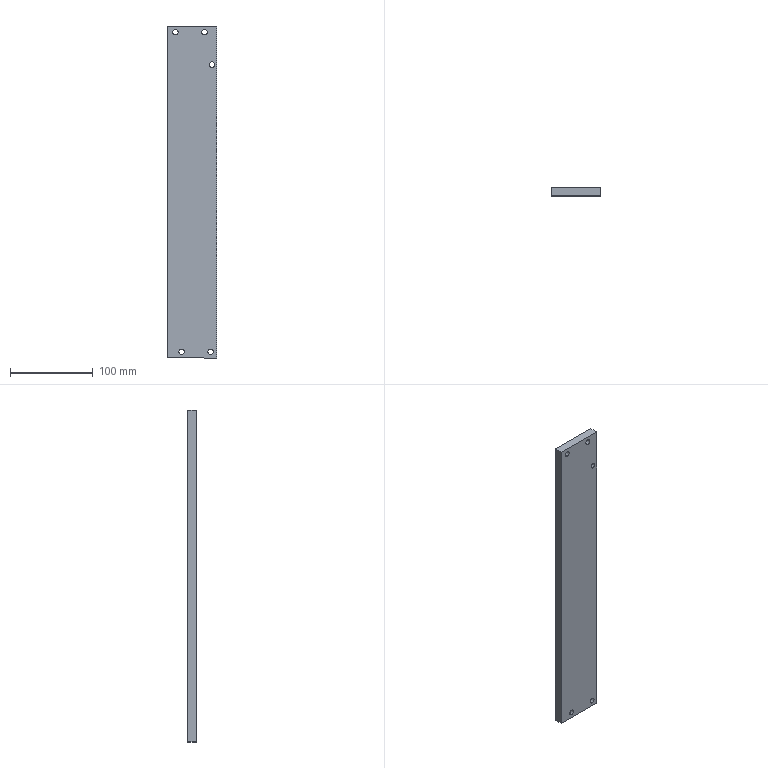Component | SolidWorks | CTM-HVS-42-02-30-1 | 1 solid | 16 faces | box 60 x 10 x 400 mm | volume 238289 mm3 | cylinder 10 | plane 6 | commonest cylinder face diameters 6.6 x10 | material Q235A
build123d program:
from build123d import *

# Parameters (mm, degrees)
SKETCH1_W                      = 400
SKETCH1_H                      = 60
EXTRUDE1_DEPTH                 = 5
SKETCH2_R                      = 3.3
EXTRUDE2_DEPTH                 = 203.485
LPATTERN1_COUNT                = 2
LPATTERN1_PITCH                = 35
M6_CLEARANCE_HOLE1_D           = 6.6
M6_CLEARANCE_HOLE1_DEPTH       = 50
M6_CLEARANCE_HOLE1_TIP         = 1.983
F_6_6_6_6_DIAMETER_HOLE1_D     = 6.6
F_6_6_6_6_DIAMETER_HOLE1_DEPTH = 30
F_6_6_6_6_DIAMETER_HOLE1_TIP   = 1.983


with BuildPart() as part:
    # Sketch1 → Extrude1 (new, symmetric)
    with BuildSketch(Plane.XY):
        Rectangle(SKETCH1_W, SKETCH1_H)
    extrude(amount=EXTRUDE1_DEPTH, both=True)

    # Sketch2 → Extrude2 (cut, through all)
    with BuildSketch(Plane.XY.offset(5)):
        with Locations((-192.5, 20)):
            Circle(SKETCH2_R)
    extrude2 = extrude(amount=-EXTRUDE2_DEPTH, mode=Mode.SUBTRACT)

    # LPattern1: Extrude2 ×2
    with Locations(*[(0, -i * LPATTERN1_PITCH, 0) for i in range(1, LPATTERN1_COUNT)]):
        add(extrude2, mode=Mode.SUBTRACT)

    # M6 Clearance Hole1
    with Locations(Plane.XY.offset(5)):
        with Locations((192.5, 12.5), (192.5, -22.5)):
            Hole(M6_CLEARANCE_HOLE1_D / 2, depth=M6_CLEARANCE_HOLE1_DEPTH)
            with Locations((0, 0, -(M6_CLEARANCE_HOLE1_DEPTH + M6_CLEARANCE_HOLE1_TIP / 2))):  # 118° drill point
                Cone(0, M6_CLEARANCE_HOLE1_D / 2, M6_CLEARANCE_HOLE1_TIP, mode=Mode.SUBTRACT)

    # 6.6 _6.6_ Diameter Hole1
    with Locations(Plane.XY.offset(5)):
        with Locations((-153.5, -24)):
            Hole(F_6_6_6_6_DIAMETER_HOLE1_D / 2, depth=F_6_6_6_6_DIAMETER_HOLE1_DEPTH)
            with Locations((0, 0, -(F_6_6_6_6_DIAMETER_HOLE1_DEPTH + F_6_6_6_6_DIAMETER_HOLE1_TIP / 2))):  # 118° drill point
                Cone(0, F_6_6_6_6_DIAMETER_HOLE1_D / 2, F_6_6_6_6_DIAMETER_HOLE1_TIP, mode=Mode.SUBTRACT)


solid = part.part

# Placed as in the assembly
solid = solid.moved(Location((-292.307, 87.443, 192.5), (-90, 0, 90)))
STEP:
#1=COLOUR_RGB('',0.7922,0.8196,0.9333);
#2=FILL_AREA_STYLE_COLOUR('',#1);
#3=FILL_AREA_STYLE('',(#2));
#4=SURFACE_STYLE_FILL_AREA(#3);
#5=SURFACE_SIDE_STYLE('',(#4));
#6=SURFACE_STYLE_USAGE(.BOTH.,#5);
#7=PRESENTATION_STYLE_ASSIGNMENT((#6));
#8=CARTESIAN_POINT('',(-10.563,3.246,13.752));
#9=VERTEX_POINT('',#8);
#10=CARTESIAN_POINT('',(-10.563,3.246,13.492));
#11=VERTEX_POINT('',#10);
#12=CARTESIAN_POINT('',(-10.563,3.246,13.622));
#13=DIRECTION('',(0.,1.,-0.));
#14=DIRECTION('',(0.,0.,-1.));
#15=AXIS2_PLACEMENT_3D('',#12,#13,#14);
#16=CIRCLE('',#15,0.1299);
#17=EDGE_CURVE('',#9,#11,#16,.T.);
#18=ORIENTED_EDGE('',*,*,#17,.F.);
#19=CARTESIAN_POINT('',(-10.563,3.639,13.752));
#20=VERTEX_POINT('',#19);
#21=CARTESIAN_POINT('',(-10.563,3.639,13.752));
#22=DIRECTION('',(0.,1.,-0.));
#23=VECTOR('',#22,39.37);
#24=LINE('',#21,#23);
#25=EDGE_CURVE('',#9,#20,#24,.T.);
#26=ORIENTED_EDGE('',*,*,#25,.T.);
#27=CARTESIAN_POINT('',(-10.563,3.639,13.492));
#28=VERTEX_POINT('',#27);
#29=CARTESIAN_POINT('',(-10.563,3.639,13.622));
#30=DIRECTION('',(0.,1.,-0.));
#31=DIRECTION('',(0.,0.,-1.));
#32=AXIS2_PLACEMENT_3D('',#29,#30,#31);
#33=CIRCLE('',#32,0.1299);
#34=EDGE_CURVE('',#20,#28,#33,.T.);
#35=ORIENTED_EDGE('',*,*,#34,.T.);
#36=CARTESIAN_POINT('',(-10.563,3.639,13.492));
#37=DIRECTION('',(0.,1.,-0.));
#38=VECTOR('',#37,39.37);
#39=LINE('',#36,#38);
#40=EDGE_CURVE('',#11,#28,#39,.T.);
#41=ORIENTED_EDGE('',*,*,#40,.F.);
#42=EDGE_LOOP('',(#18,#26,#35,#41));
#43=FACE_OUTER_BOUND('',#42,.T.);
#44=CARTESIAN_POINT('',(-10.563,3.639,13.622));
#45=DIRECTION('',(0.,1.,-0.));
#46=DIRECTION('',(0.,0.,-1.));
#47=AXIS2_PLACEMENT_3D('',#44,#45,#46);
#48=CYLINDRICAL_SURFACE('',#47,0.1299);
#49=ADVANCED_FACE('',(#43),#48,.F.);
#50=CARTESIAN_POINT('',(-12.,3.246,0.1299));
#51=VERTEX_POINT('',#50);
#52=CARTESIAN_POINT('',(-12.,3.246,-0.1299));
#53=VERTEX_POINT('',#52);
#54=CARTESIAN_POINT('',(-12.,3.246,0.));
#55=DIRECTION('',(0.,1.,-0.));
#56=DIRECTION('',(0.,0.,-1.));
#57=AXIS2_PLACEMENT_3D('',#54,#55,#56);
#58=CIRCLE('',#57,0.1299);
#59=EDGE_CURVE('',#51,#53,#58,.T.);
#60=ORIENTED_EDGE('',*,*,#59,.F.);
#61=CARTESIAN_POINT('',(-12.,3.639,0.1299));
#62=VERTEX_POINT('',#61);
#63=CARTESIAN_POINT('',(-12.,3.639,0.1299));
#64=DIRECTION('',(0.,1.,-0.));
#65=VECTOR('',#64,39.37);
#66=LINE('',#63,#65);
#67=EDGE_CURVE('',#51,#62,#66,.T.);
#68=ORIENTED_EDGE('',*,*,#67,.T.);
#69=CARTESIAN_POINT('',(-12.,3.639,-0.1299));
#70=VERTEX_POINT('',#69);
#71=CARTESIAN_POINT('',(-12.,3.639,0.));
#72=DIRECTION('',(0.,1.,-0.));
#73=DIRECTION('',(0.,0.,-1.));
#74=AXIS2_PLACEMENT_3D('',#71,#72,#73);
#75=CIRCLE('',#74,0.1299);
#76=EDGE_CURVE('',#62,#70,#75,.T.);
#77=ORIENTED_EDGE('',*,*,#76,.T.);
#78=CARTESIAN_POINT('',(-12.,3.639,-0.1299));
#79=DIRECTION('',(0.,1.,-0.));
#80=VECTOR('',#79,39.37);
#81=LINE('',#78,#80);
#82=EDGE_CURVE('',#53,#70,#81,.T.);
#83=ORIENTED_EDGE('',*,*,#82,.F.);
#84=EDGE_LOOP('',(#60,#68,#77,#83));
#85=FACE_OUTER_BOUND('',#84,.T.);
#86=CARTESIAN_POINT('',(-12.,3.639,0.));
#87=DIRECTION('',(0.,1.,-0.));
#88=DIRECTION('',(0.,0.,-1.));
#89=AXIS2_PLACEMENT_3D('',#86,#87,#88);
#90=CYLINDRICAL_SURFACE('',#89,0.1299);
#91=ADVANCED_FACE('',(#85),#90,.F.);
#92=CARTESIAN_POINT('',(-10.622,3.246,0.1299));
#93=VERTEX_POINT('',#92);
#94=CARTESIAN_POINT('',(-10.622,3.246,-0.1299));
#95=VERTEX_POINT('',#94);
#96=CARTESIAN_POINT('',(-10.622,3.246,0.));
#97=DIRECTION('',(0.,1.,-0.));
#98=DIRECTION('',(0.,0.,-1.));
#99=AXIS2_PLACEMENT_3D('',#96,#97,#98);
#100=CIRCLE('',#99,0.1299);
#101=EDGE_CURVE('',#93,#95,#100,.T.);
#102=ORIENTED_EDGE('',*,*,#101,.F.);
#103=CARTESIAN_POINT('',(-10.622,3.639,0.1299));
#104=VERTEX_POINT('',#103);
#105=CARTESIAN_POINT('',(-10.622,3.639,0.1299));
#106=DIRECTION('',(0.,1.,-0.));
#107=VECTOR('',#106,39.37);
#108=LINE('',#105,#107);
#109=EDGE_CURVE('',#93,#104,#108,.T.);
#110=ORIENTED_EDGE('',*,*,#109,.T.);
#111=CARTESIAN_POINT('',(-10.622,3.639,-0.1299));
#112=VERTEX_POINT('',#111);
#113=CARTESIAN_POINT('',(-10.622,3.639,0.));
#114=DIRECTION('',(0.,1.,-0.));
#115=DIRECTION('',(0.,0.,-1.));
#116=AXIS2_PLACEMENT_3D('',#113,#114,#115);
#117=CIRCLE('',#116,0.1299);
#118=EDGE_CURVE('',#104,#112,#117,.T.);
#119=ORIENTED_EDGE('',*,*,#118,.T.);
#120=CARTESIAN_POINT('',(-10.622,3.639,-0.1299));
#121=DIRECTION('',(0.,1.,-0.));
#122=VECTOR('',#121,39.37);
#123=LINE('',#120,#122);
#124=EDGE_CURVE('',#95,#112,#123,.T.);
#125=ORIENTED_EDGE('',*,*,#124,.F.);
#126=EDGE_LOOP('',(#102,#110,#119,#125));
#127=FACE_OUTER_BOUND('',#126,.T.);
#128=CARTESIAN_POINT('',(-10.622,3.639,0.));
#129=DIRECTION('',(0.,1.,-0.));
#130=DIRECTION('',(0.,0.,-1.));
#131=AXIS2_PLACEMENT_3D('',#128,#129,#130);
#132=CYLINDRICAL_SURFACE('',#131,0.1299);
#133=ADVANCED_FACE('',(#127),#132,.F.);
#134=CARTESIAN_POINT('',(-10.918,3.246,15.287));
#135=VERTEX_POINT('',#134);
#136=CARTESIAN_POINT('',(-10.918,3.246,15.028));
#137=VERTEX_POINT('',#136);
#138=CARTESIAN_POINT('',(-10.918,3.246,15.157));
#139=DIRECTION('',(0.,1.,-0.));
#140=DIRECTION('',(0.,0.,-1.));
#141=AXIS2_PLACEMENT_3D('',#138,#139,#140);
#142=CIRCLE('',#141,0.1299);
#143=EDGE_CURVE('',#135,#137,#142,.T.);
#144=ORIENTED_EDGE('',*,*,#143,.F.);
#145=CARTESIAN_POINT('',(-10.918,3.639,15.287));
#146=VERTEX_POINT('',#145);
#147=CARTESIAN_POINT('',(-10.918,3.246,15.287));
#148=DIRECTION('',(0.,1.,-0.));
#149=VECTOR('',#148,39.37);
#150=LINE('',#147,#149);
#151=EDGE_CURVE('',#135,#146,#150,.T.);
#152=ORIENTED_EDGE('',*,*,#151,.T.);
#153=CARTESIAN_POINT('',(-10.918,3.639,15.028));
#154=VERTEX_POINT('',#153);
#155=CARTESIAN_POINT('',(-10.918,3.639,15.157));
#156=DIRECTION('',(0.,1.,-0.));
#157=DIRECTION('',(0.,0.,-1.));
#158=AXIS2_PLACEMENT_3D('',#155,#156,#157);
#159=CIRCLE('',#158,0.1299);
#160=EDGE_CURVE('',#146,#154,#159,.T.);
#161=ORIENTED_EDGE('',*,*,#160,.T.);
#162=CARTESIAN_POINT('',(-10.918,3.246,15.028));
#163=DIRECTION('',(0.,1.,-0.));
#164=VECTOR('',#163,39.37);
#165=LINE('',#162,#164);
#166=EDGE_CURVE('',#137,#154,#165,.T.);
#167=ORIENTED_EDGE('',*,*,#166,.F.);
#168=EDGE_LOOP('',(#144,#152,#161,#167));
#169=FACE_OUTER_BOUND('',#168,.T.);
#170=CARTESIAN_POINT('',(-10.918,3.246,15.157));
#171=DIRECTION('',(0.,1.,-0.));
#172=DIRECTION('',(0.,0.,-1.));
#173=AXIS2_PLACEMENT_3D('',#170,#171,#172);
#174=CYLINDRICAL_SURFACE('',#173,0.1299);
#175=ADVANCED_FACE('',(#169),#174,.F.);
#176=CARTESIAN_POINT('',(-12.296,3.246,15.287));
#177=VERTEX_POINT('',#176);
#178=CARTESIAN_POINT('',(-12.296,3.246,15.028));
#179=VERTEX_POINT('',#178);
#180=CARTESIAN_POINT('',(-12.296,3.246,15.157));
#181=DIRECTION('',(0.,1.,-0.));
#182=DIRECTION('',(0.,0.,-1.));
#183=AXIS2_PLACEMENT_3D('',#180,#181,#182);
#184=CIRCLE('',#183,0.1299);
#185=EDGE_CURVE('',#177,#179,#184,.T.);
#186=ORIENTED_EDGE('',*,*,#185,.F.);
#187=CARTESIAN_POINT('',(-12.296,3.639,15.287));
#188=VERTEX_POINT('',#187);
#189=CARTESIAN_POINT('',(-12.296,3.246,15.287));
#190=DIRECTION('',(0.,1.,-0.));
#191=VECTOR('',#190,39.37);
#192=LINE('',#189,#191);
#193=EDGE_CURVE('',#177,#188,#192,.T.);
#194=ORIENTED_EDGE('',*,*,#193,.T.);
#195=CARTESIAN_POINT('',(-12.296,3.639,15.028));
#196=VERTEX_POINT('',#195);
#197=CARTESIAN_POINT('',(-12.296,3.639,15.157));
#198=DIRECTION('',(0.,1.,-0.));
#199=DIRECTION('',(0.,0.,-1.));
#200=AXIS2_PLACEMENT_3D('',#197,#198,#199);
#201=CIRCLE('',#200,0.1299);
#202=EDGE_CURVE('',#188,#196,#201,.T.);
#203=ORIENTED_EDGE('',*,*,#202,.T.);
#204=CARTESIAN_POINT('',(-12.296,3.246,15.028));
#205=DIRECTION('',(0.,1.,-0.));
#206=VECTOR('',#205,39.37);
#207=LINE('',#204,#206);
#208=EDGE_CURVE('',#179,#196,#207,.T.);
#209=ORIENTED_EDGE('',*,*,#208,.F.);
#210=EDGE_LOOP('',(#186,#194,#203,#209));
#211=FACE_OUTER_BOUND('',#210,.T.);
#212=CARTESIAN_POINT('',(-12.296,3.246,15.157));
#213=DIRECTION('',(0.,1.,-0.));
#214=DIRECTION('',(0.,0.,-1.));
#215=AXIS2_PLACEMENT_3D('',#212,#213,#214);
#216=CYLINDRICAL_SURFACE('',#215,0.1299);
#217=ADVANCED_FACE('',(#211),#216,.F.);
#218=CARTESIAN_POINT('',(-10.327,3.246,-0.2953));
#219=VERTEX_POINT('',#218);
#220=CARTESIAN_POINT('',(-12.689,3.246,-0.2953));
#221=VERTEX_POINT('',#220);
#222=CARTESIAN_POINT('',(-12.689,3.246,-0.2953));
#223=DIRECTION('',(-1.,0.,0.));
#224=VECTOR('',#223,39.37);
#225=LINE('',#222,#224);
#226=EDGE_CURVE('',#219,#221,#225,.T.);
#227=ORIENTED_EDGE('',*,*,#226,.T.);
#228=CARTESIAN_POINT('',(-12.689,3.639,-0.2953));
#229=VERTEX_POINT('',#228);
#230=CARTESIAN_POINT('',(-12.689,3.639,-0.2953));
#231=DIRECTION('',(-0.,-1.,0.));
#232=VECTOR('',#231,39.37);
#233=LINE('',#230,#232);
#234=EDGE_CURVE('',#229,#221,#233,.T.);
#235=ORIENTED_EDGE('',*,*,#234,.F.);
#236=CARTESIAN_POINT('',(-10.327,3.639,-0.2953));
#237=VERTEX_POINT('',#236);
#238=CARTESIAN_POINT('',(-12.689,3.639,-0.2953));
#239=DIRECTION('',(-1.,0.,0.));
#240=VECTOR('',#239,39.37);
#241=LINE('',#238,#240);
#242=EDGE_CURVE('',#237,#229,#241,.T.);
#243=ORIENTED_EDGE('',*,*,#242,.F.);
#244=CARTESIAN_POINT('',(-10.327,3.639,-0.2953));
#245=DIRECTION('',(-0.,-1.,0.));
#246=VECTOR('',#245,39.37);
#247=LINE('',#244,#246);
#248=EDGE_CURVE('',#237,#219,#247,.T.);
#249=ORIENTED_EDGE('',*,*,#248,.T.);
#250=EDGE_LOOP('',(#227,#235,#243,#249));
#251=FACE_OUTER_BOUND('',#250,.T.);
#252=CARTESIAN_POINT('',(-12.689,3.639,-0.2953));
#253=DIRECTION('',(0.,0.,1.));
#254=DIRECTION('',(0.,1.,-0.));
#255=AXIS2_PLACEMENT_3D('',#252,#253,#254);
#256=PLANE('',#255);
#257=ADVANCED_FACE('',(#251),#256,.F.);
#258=CARTESIAN_POINT('',(-12.689,3.246,15.453));
#259=VERTEX_POINT('',#258);
#260=CARTESIAN_POINT('',(-12.689,3.246,15.453));
#261=DIRECTION('',(0.,0.,1.));
#262=VECTOR('',#261,39.37);
#263=LINE('',#260,#262);
#264=EDGE_CURVE('',#221,#259,#263,.T.);
#265=ORIENTED_EDGE('',*,*,#264,.T.);
#266=CARTESIAN_POINT('',(-12.689,3.639,15.453));
#267=VERTEX_POINT('',#266);
#268=CARTESIAN_POINT('',(-12.689,3.639,15.453));
#269=DIRECTION('',(-0.,-1.,0.));
#270=VECTOR('',#269,39.37);
#271=LINE('',#268,#270);
#272=EDGE_CURVE('',#267,#259,#271,.T.);
#273=ORIENTED_EDGE('',*,*,#272,.F.);
#274=CARTESIAN_POINT('',(-12.689,3.639,15.453));
#275=DIRECTION('',(0.,0.,1.));
#276=VECTOR('',#275,39.37);
#277=LINE('',#274,#276);
#278=EDGE_CURVE('',#229,#267,#277,.T.);
#279=ORIENTED_EDGE('',*,*,#278,.F.);
#280=ORIENTED_EDGE('',*,*,#234,.T.);
#281=EDGE_LOOP('',(#265,#273,#279,#280));
#282=FACE_OUTER_BOUND('',#281,.T.);
#283=CARTESIAN_POINT('',(-12.689,3.639,15.453));
#284=DIRECTION('',(1.,-0.,-0.));
#285=DIRECTION('',(-0.,-1.,0.));
#286=AXIS2_PLACEMENT_3D('',#283,#284,#285);
#287=PLANE('',#286);
#288=ADVANCED_FACE('',(#282),#287,.F.);
#289=CARTESIAN_POINT('',(-10.327,3.246,15.453));
#290=VERTEX_POINT('',#289);
#291=CARTESIAN_POINT('',(-12.689,3.246,15.453));
#292=DIRECTION('',(1.,-0.,-0.));
#293=VECTOR('',#292,39.37);
#294=LINE('',#291,#293);
#295=EDGE_CURVE('',#259,#290,#294,.T.);
#296=ORIENTED_EDGE('',*,*,#295,.T.);
#297=CARTESIAN_POINT('',(-10.327,3.639,15.453));
#298=VERTEX_POINT('',#297);
#299=CARTESIAN_POINT('',(-10.327,3.639,15.453));
#300=DIRECTION('',(-0.,-1.,0.));
#301=VECTOR('',#300,39.37);
#302=LINE('',#299,#301);
#303=EDGE_CURVE('',#298,#290,#302,.T.);
#304=ORIENTED_EDGE('',*,*,#303,.F.);
#305=CARTESIAN_POINT('',(-12.689,3.639,15.453));
#306=DIRECTION('',(1.,-0.,-0.));
#307=VECTOR('',#306,39.37);
#308=LINE('',#305,#307);
#309=EDGE_CURVE('',#267,#298,#308,.T.);
#310=ORIENTED_EDGE('',*,*,#309,.F.);
#311=ORIENTED_EDGE('',*,*,#272,.T.);
#312=EDGE_LOOP('',(#296,#304,#310,#311));
#313=FACE_OUTER_BOUND('',#312,.T.);
#314=CARTESIAN_POINT('',(-12.689,3.639,15.453));
#315=DIRECTION('',(-0.,-0.,-1.));
#316=DIRECTION('',(-0.,-1.,0.));
#317=AXIS2_PLACEMENT_3D('',#314,#315,#316);
#318=PLANE('',#317);
#319=ADVANCED_FACE('',(#313),#318,.F.);
#320=CARTESIAN_POINT('',(-10.327,3.246,15.453));
#321=DIRECTION('',(-0.,-0.,-1.));
#322=VECTOR('',#321,39.37);
#323=LINE('',#320,#322);
#324=EDGE_CURVE('',#290,#219,#323,.T.);
#325=ORIENTED_EDGE('',*,*,#324,.T.);
#326=ORIENTED_EDGE('',*,*,#248,.F.);
#327=CARTESIAN_POINT('',(-10.327,3.639,15.453));
#328=DIRECTION('',(-0.,-0.,-1.));
#329=VECTOR('',#328,39.37);
#330=LINE('',#327,#329);
#331=EDGE_CURVE('',#298,#237,#330,.T.);
#332=ORIENTED_EDGE('',*,*,#331,.F.);
#333=ORIENTED_EDGE('',*,*,#303,.T.);
#334=EDGE_LOOP('',(#325,#326,#332,#333));
#335=FACE_OUTER_BOUND('',#334,.T.);
#336=CARTESIAN_POINT('',(-10.327,3.639,15.453));
#337=DIRECTION('',(-1.,0.,0.));
#338=DIRECTION('',(0.,1.,-0.));
#339=AXIS2_PLACEMENT_3D('',#336,#337,#338);
#340=PLANE('',#339);
#341=ADVANCED_FACE('',(#335),#340,.F.);
#342=CARTESIAN_POINT('',(-10.563,3.639,13.622));
#343=DIRECTION('',(0.,1.,-0.));
#344=DIRECTION('',(0.,0.,-1.));
#345=AXIS2_PLACEMENT_3D('',#342,#343,#344);
#346=CIRCLE('',#345,0.1299);
#347=EDGE_CURVE('',#28,#20,#346,.T.);
#348=ORIENTED_EDGE('',*,*,#347,.F.);
#349=ORIENTED_EDGE('',*,*,#34,.F.);
#350=EDGE_LOOP('',(#348,#349));
#351=FACE_BOUND('',#350,.T.);
#352=CARTESIAN_POINT('',(-12.,3.639,0.));
#353=DIRECTION('',(0.,1.,-0.));
#354=DIRECTION('',(0.,0.,-1.));
#355=AXIS2_PLACEMENT_3D('',#352,#353,#354);
#356=CIRCLE('',#355,0.1299);
#357=EDGE_CURVE('',#70,#62,#356,.T.);
#358=ORIENTED_EDGE('',*,*,#357,.F.);
#359=ORIENTED_EDGE('',*,*,#76,.F.);
#360=EDGE_LOOP('',(#358,#359));
#361=FACE_BOUND('',#360,.T.);
#362=CARTESIAN_POINT('',(-10.622,3.639,0.));
#363=DIRECTION('',(0.,1.,-0.));
#364=DIRECTION('',(0.,0.,-1.));
#365=AXIS2_PLACEMENT_3D('',#362,#363,#364);
#366=CIRCLE('',#365,0.1299);
#367=EDGE_CURVE('',#112,#104,#366,.T.);
#368=ORIENTED_EDGE('',*,*,#367,.F.);
#369=ORIENTED_EDGE('',*,*,#118,.F.);
#370=EDGE_LOOP('',(#368,#369));
#371=FACE_BOUND('',#370,.T.);
#372=CARTESIAN_POINT('',(-10.918,3.639,15.157));
#373=DIRECTION('',(0.,1.,-0.));
#374=DIRECTION('',(0.,0.,-1.));
#375=AXIS2_PLACEMENT_3D('',#372,#373,#374);
#376=CIRCLE('',#375,0.1299);
#377=EDGE_CURVE('',#154,#146,#376,.T.);
#378=ORIENTED_EDGE('',*,*,#377,.F.);
#379=ORIENTED_EDGE('',*,*,#160,.F.);
#380=EDGE_LOOP('',(#378,#379));
#381=FACE_BOUND('',#380,.T.);
#382=CARTESIAN_POINT('',(-12.296,3.639,15.157));
#383=DIRECTION('',(0.,1.,-0.));
#384=DIRECTION('',(0.,0.,-1.));
#385=AXIS2_PLACEMENT_3D('',#382,#383,#384);
#386=CIRCLE('',#385,0.1299);
#387=EDGE_CURVE('',#196,#188,#386,.T.);
#388=ORIENTED_EDGE('',*,*,#387,.F.);
#389=ORIENTED_EDGE('',*,*,#202,.F.);
#390=EDGE_LOOP('',(#388,#389));
#391=FACE_BOUND('',#390,.T.);
#392=ORIENTED_EDGE('',*,*,#242,.T.);
#393=ORIENTED_EDGE('',*,*,#278,.T.);
#394=ORIENTED_EDGE('',*,*,#309,.T.);
#395=ORIENTED_EDGE('',*,*,#331,.T.);
#396=EDGE_LOOP('',(#392,#393,#394,#395));
#397=FACE_OUTER_BOUND('',#396,.T.);
#398=CARTESIAN_POINT('',(-10.327,3.639,-0.2953));
#399=DIRECTION('',(0.,1.,-0.));
#400=DIRECTION('',(-0.,-0.,-1.));
#401=AXIS2_PLACEMENT_3D('',#398,#399,#400);
#402=PLANE('',#401);
#403=ADVANCED_FACE('',(#351,#361,#371,#381,#391,#397),#402,.T.);
#404=CARTESIAN_POINT('',(-10.563,3.246,13.622));
#405=DIRECTION('',(0.,1.,-0.));
#406=DIRECTION('',(0.,0.,-1.));
#407=AXIS2_PLACEMENT_3D('',#404,#405,#406);
#408=CIRCLE('',#407,0.1299);
#409=EDGE_CURVE('',#11,#9,#408,.T.);
#410=ORIENTED_EDGE('',*,*,#409,.T.);
#411=ORIENTED_EDGE('',*,*,#17,.T.);
#412=EDGE_LOOP('',(#410,#411));
#413=FACE_BOUND('',#412,.T.);
#414=CARTESIAN_POINT('',(-12.,3.246,0.));
#415=DIRECTION('',(0.,1.,-0.));
#416=DIRECTION('',(0.,0.,-1.));
#417=AXIS2_PLACEMENT_3D('',#414,#415,#416);
#418=CIRCLE('',#417,0.1299);
#419=EDGE_CURVE('',#53,#51,#418,.T.);
#420=ORIENTED_EDGE('',*,*,#419,.T.);
#421=ORIENTED_EDGE('',*,*,#59,.T.);
#422=EDGE_LOOP('',(#420,#421));
#423=FACE_BOUND('',#422,.T.);
#424=CARTESIAN_POINT('',(-10.622,3.246,0.));
#425=DIRECTION('',(0.,1.,-0.));
#426=DIRECTION('',(0.,0.,-1.));
#427=AXIS2_PLACEMENT_3D('',#424,#425,#426);
#428=CIRCLE('',#427,0.1299);
#429=EDGE_CURVE('',#95,#93,#428,.T.);
#430=ORIENTED_EDGE('',*,*,#429,.T.);
#431=ORIENTED_EDGE('',*,*,#101,.T.);
#432=EDGE_LOOP('',(#430,#431));
#433=FACE_BOUND('',#432,.T.);
#434=CARTESIAN_POINT('',(-10.918,3.246,15.157));
#435=DIRECTION('',(0.,1.,-0.));
#436=DIRECTION('',(0.,0.,-1.));
#437=AXIS2_PLACEMENT_3D('',#434,#435,#436);
#438=CIRCLE('',#437,0.1299);
#439=EDGE_CURVE('',#137,#135,#438,.T.);
#440=ORIENTED_EDGE('',*,*,#439,.T.);
#441=ORIENTED_EDGE('',*,*,#143,.T.);
#442=EDGE_LOOP('',(#440,#441));
#443=FACE_BOUND('',#442,.T.);
#444=CARTESIAN_POINT('',(-12.296,3.246,15.157));
#445=DIRECTION('',(0.,1.,-0.));
#446=DIRECTION('',(0.,0.,-1.));
#447=AXIS2_PLACEMENT_3D('',#444,#445,#446);
#448=CIRCLE('',#447,0.1299);
#449=EDGE_CURVE('',#179,#177,#448,.T.);
#450=ORIENTED_EDGE('',*,*,#449,.T.);
#451=ORIENTED_EDGE('',*,*,#185,.T.);
#452=EDGE_LOOP('',(#450,#451));
#453=FACE_BOUND('',#452,.T.);
#454=ORIENTED_EDGE('',*,*,#226,.F.);
#455=ORIENTED_EDGE('',*,*,#324,.F.);
#456=ORIENTED_EDGE('',*,*,#295,.F.);
#457=ORIENTED_EDGE('',*,*,#264,.F.);
#458=EDGE_LOOP('',(#454,#455,#456,#457));
#459=FACE_OUTER_BOUND('',#458,.T.);
#460=CARTESIAN_POINT('',(-10.327,3.246,-0.2953));
#461=DIRECTION('',(0.,1.,-0.));
#462=DIRECTION('',(-0.,-0.,-1.));
#463=AXIS2_PLACEMENT_3D('',#460,#461,#462);
#464=PLANE('',#463);
#465=ADVANCED_FACE('',(#413,#423,#433,#443,#453,#459),#464,.F.);
#466=ORIENTED_EDGE('',*,*,#193,.F.);
#467=ORIENTED_EDGE('',*,*,#449,.F.);
#468=ORIENTED_EDGE('',*,*,#208,.T.);
#469=ORIENTED_EDGE('',*,*,#387,.T.);
#470=EDGE_LOOP('',(#466,#467,#468,#469));
#471=FACE_OUTER_BOUND('',#470,.T.);
#472=CARTESIAN_POINT('',(-12.296,3.246,15.157));
#473=DIRECTION('',(0.,1.,-0.));
#474=DIRECTION('',(0.,0.,-1.));
#475=AXIS2_PLACEMENT_3D('',#472,#473,#474);
#476=CYLINDRICAL_SURFACE('',#475,0.1299);
#477=ADVANCED_FACE('',(#471),#476,.F.);
#478=ORIENTED_EDGE('',*,*,#151,.F.);
#479=ORIENTED_EDGE('',*,*,#439,.F.);
#480=ORIENTED_EDGE('',*,*,#166,.T.);
#481=ORIENTED_EDGE('',*,*,#377,.T.);
#482=EDGE_LOOP('',(#478,#479,#480,#481));
#483=FACE_OUTER_BOUND('',#482,.T.);
#484=CARTESIAN_POINT('',(-10.918,3.246,15.157));
#485=DIRECTION('',(0.,1.,-0.));
#486=DIRECTION('',(0.,0.,-1.));
#487=AXIS2_PLACEMENT_3D('',#484,#485,#486);
#488=CYLINDRICAL_SURFACE('',#487,0.1299);
#489=ADVANCED_FACE('',(#483),#488,.F.);
#490=ORIENTED_EDGE('',*,*,#109,.F.);
#491=ORIENTED_EDGE('',*,*,#429,.F.);
#492=ORIENTED_EDGE('',*,*,#124,.T.);
#493=ORIENTED_EDGE('',*,*,#367,.T.);
#494=EDGE_LOOP('',(#490,#491,#492,#493));
#495=FACE_OUTER_BOUND('',#494,.T.);
#496=CARTESIAN_POINT('',(-10.622,3.639,0.));
#497=DIRECTION('',(0.,1.,-0.));
#498=DIRECTION('',(0.,0.,-1.));
#499=AXIS2_PLACEMENT_3D('',#496,#497,#498);
#500=CYLINDRICAL_SURFACE('',#499,0.1299);
#501=ADVANCED_FACE('',(#495),#500,.F.);
#502=ORIENTED_EDGE('',*,*,#67,.F.);
#503=ORIENTED_EDGE('',*,*,#419,.F.);
#504=ORIENTED_EDGE('',*,*,#82,.T.);
#505=ORIENTED_EDGE('',*,*,#357,.T.);
#506=EDGE_LOOP('',(#502,#503,#504,#505));
#507=FACE_OUTER_BOUND('',#506,.T.);
#508=CARTESIAN_POINT('',(-12.,3.639,0.));
#509=DIRECTION('',(0.,1.,-0.));
#510=DIRECTION('',(0.,0.,-1.));
#511=AXIS2_PLACEMENT_3D('',#508,#509,#510);
#512=CYLINDRICAL_SURFACE('',#511,0.1299);
#513=ADVANCED_FACE('',(#507),#512,.F.);
#514=ORIENTED_EDGE('',*,*,#25,.F.);
#515=ORIENTED_EDGE('',*,*,#409,.F.);
#516=ORIENTED_EDGE('',*,*,#40,.T.);
#517=ORIENTED_EDGE('',*,*,#347,.T.);
#518=EDGE_LOOP('',(#514,#515,#516,#517));
#519=FACE_OUTER_BOUND('',#518,.T.);
#520=CARTESIAN_POINT('',(-10.563,3.639,13.622));
#521=DIRECTION('',(0.,1.,-0.));
#522=DIRECTION('',(0.,0.,-1.));
#523=AXIS2_PLACEMENT_3D('',#520,#521,#522);
#524=CYLINDRICAL_SURFACE('',#523,0.1299);
#525=ADVANCED_FACE('',(#519),#524,.F.);
#526=CLOSED_SHELL('',(#49,#91,#133,#175,#217,#257,#288,#319,#341,#403,#465,#477,#489,#501,#513,#525));
#527=MANIFOLD_SOLID_BREP('',#526);
#528=STYLED_ITEM('',(#7),#527);
#529=PRESENTATION_LAYER_ASSIGNMENT('','',(#528));
#530=(LENGTH_UNIT()NAMED_UNIT(*)SI_UNIT($,.METRE.));
#531=LENGTH_MEASURE_WITH_UNIT(LENGTH_MEASURE(0.0254),#530);
#532=DIMENSIONAL_EXPONENTS(1.,0.,0.,0.,0.,0.,0.);
#533=(CONVERSION_BASED_UNIT('',#531)LENGTH_UNIT()NAMED_UNIT(#532));
#534=UNCERTAINTY_MEASURE_WITH_UNIT(LENGTH_MEASURE(0.00001),#533,'','');
#535=(NAMED_UNIT(*)PLANE_ANGLE_UNIT()SI_UNIT($,.RADIAN.));
#536=(NAMED_UNIT(*)SI_UNIT($,.STERADIAN.)SOLID_ANGLE_UNIT());
#537=(GEOMETRIC_REPRESENTATION_CONTEXT(3)GLOBAL_UNCERTAINTY_ASSIGNED_CONTEXT((#534))GLOBAL_UNIT_ASSIGNED_CONTEXT((#533,#535,#536))REPRESENTATION_CONTEXT('',''));
#538=MECHANICAL_DESIGN_GEOMETRIC_PRESENTATION_REPRESENTATION('',(#528),#537);
#539=CARTESIAN_POINT('',(0.,0.,0.));
#540=DIRECTION('',(0.,0.,1.));
#541=DIRECTION('',(1.,0.,0.));
#542=AXIS2_PLACEMENT_3D('',#539,#540,#541);
#543=(LENGTH_UNIT()NAMED_UNIT(*)SI_UNIT($,.METRE.));
#544=LENGTH_MEASURE_WITH_UNIT(LENGTH_MEASURE(0.0254),#543);
#545=DIMENSIONAL_EXPONENTS(1.,0.,0.,0.,0.,0.,0.);
#546=(CONVERSION_BASED_UNIT('',#544)LENGTH_UNIT()NAMED_UNIT(#545));
#547=UNCERTAINTY_MEASURE_WITH_UNIT(LENGTH_MEASURE(0.00001),#546,'','');
#548=(NAMED_UNIT(*)PLANE_ANGLE_UNIT()SI_UNIT($,.RADIAN.));
#549=(NAMED_UNIT(*)SI_UNIT($,.STERADIAN.)SOLID_ANGLE_UNIT());
#550=(GEOMETRIC_REPRESENTATION_CONTEXT(3)GLOBAL_UNCERTAINTY_ASSIGNED_CONTEXT((#547))GLOBAL_UNIT_ASSIGNED_CONTEXT((#546,#548,#549))REPRESENTATION_CONTEXT('',''));
#551=ADVANCED_BREP_SHAPE_REPRESENTATION('',(#527,#542),#550);